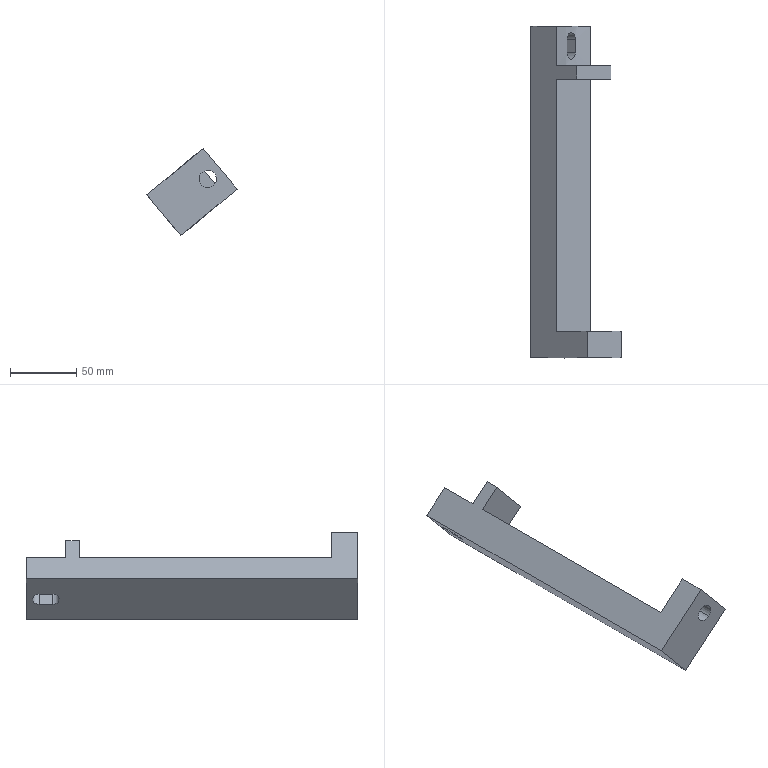Component | SolidWorks | K51-2_K51-5-2 | 1 solid | 18 faces | box 67.87 x 250 x 65.92 mm | volume 273386 mm3 | plane 13 | cylinder 5 | commonest cylinder face diameters 13 x2 10 x2 170 x1
build123d program:
from build123d import *

# Parameters (mm, degrees)
BOSS_EXTRUDE1_DEPTH = 20
SKETCH2_R           = 6.5
CUT_EXTRUDE1_DEPTH  = 30
SKETCH3_W           = 40
SKETCH3_H           = 10
BOSS_EXTRUDE2_DEPTH = 20
SKETCH4_R           = 85
CUT_EXTRUDE2_DEPTH  = 30
CUT_EXTRUDE3_DEPTH  = 30


with BuildPart() as part:
    # Sketch1 → Boss-Extrude1 (new, symmetric)
    with BuildSketch(Plane.XY):
        Polygon((0, 0), (0, 250), (25, 250), (25, 20), (55, 20), (55, 0), align=None)
    extrude(amount=BOSS_EXTRUDE1_DEPTH, both=True)

    # Sketch2 → Cut-Extrude1 (cut)
    with BuildSketch(Plane(origin=(0, 20, 0), x_dir=(1, 0, 0), z_dir=(0, 1, 0))):
        with Locations(Location((43, 0, 0), (0, 0, 270))):
            Circle(SKETCH2_R)
    extrude(amount=-CUT_EXTRUDE1_DEPTH, mode=Mode.SUBTRACT)

    # Sketch3 → Boss-Extrude2 (add)
    with BuildSketch(Plane(origin=(25, 0, 0), x_dir=(0, 0, -1), z_dir=(1, 0, 0))):
        with Locations((0, 215)):
            Rectangle(SKETCH3_W, SKETCH3_H)
    extrude(amount=BOSS_EXTRUDE2_DEPTH)

    # Sketch4 → Cut-Extrude2 (cut)
    with BuildSketch(Plane(origin=(0, 250, 0), x_dir=(1, 0, 0), z_dir=(0, 1, 0))):
        with Locations((107.614, 0)):
            Circle(SKETCH4_R)
    extrude(amount=-CUT_EXTRUDE2_DEPTH, mode=Mode.SUBTRACT)

    # Sketch5 → Cut-Extrude3 (cut)
    with BuildSketch(Plane.ZY):
        with BuildLine():
            Line((5, 240), (5, 230))
            ThreePointArc((5, 230), (0, 225), (-5, 230))
            Line((-5, 230), (-5, 240))
            ThreePointArc((-5, 240), (0, 245), (5, 240))
        make_face()
    extrude(amount=-CUT_EXTRUDE3_DEPTH, mode=Mode.SUBTRACT)


solid = part.part

# Placed as in the assembly
solid = solid.moved(Location((-338.347, 1052, 8.26), (0, -39.731, 0)))
STEP:
#1=COLOUR_RGB('',0.7922,0.8196,0.9333);
#2=FILL_AREA_STYLE_COLOUR('',#1);
#3=FILL_AREA_STYLE('',(#2));
#4=SURFACE_STYLE_FILL_AREA(#3);
#5=SURFACE_SIDE_STYLE('',(#4));
#6=SURFACE_STYLE_USAGE(.BOTH.,#5);
#7=PRESENTATION_STYLE_ASSIGNMENT((#6));
#8=CARTESIAN_POINT('',(-11.855,41.417,1.21));
#9=VERTEX_POINT('',#8);
#10=CARTESIAN_POINT('',(-12.182,41.417,1.604));
#11=VERTEX_POINT('',#10);
#12=CARTESIAN_POINT('',(-12.019,41.417,1.407));
#13=DIRECTION('',(-0.,1.,-0.));
#14=DIRECTION('',(-0.769,0.,-0.6392));
#15=AXIS2_PLACEMENT_3D('',#12,#13,#14);
#16=CIRCLE('',#15,0.2559);
#17=EDGE_CURVE('',#9,#11,#16,.T.);
#18=ORIENTED_EDGE('',*,*,#17,.F.);
#19=CARTESIAN_POINT('',(-11.855,42.205,1.21));
#20=VERTEX_POINT('',#19);
#21=CARTESIAN_POINT('',(-11.855,41.024,1.21));
#22=DIRECTION('',(-0.,1.,-0.));
#23=VECTOR('',#22,39.37);
#24=LINE('',#21,#23);
#25=EDGE_CURVE('',#9,#20,#24,.T.);
#26=ORIENTED_EDGE('',*,*,#25,.T.);
#27=CARTESIAN_POINT('',(-12.182,42.205,1.604));
#28=VERTEX_POINT('',#27);
#29=CARTESIAN_POINT('',(-12.019,42.205,1.407));
#30=DIRECTION('',(-0.,1.,-0.));
#31=DIRECTION('',(-0.6392,0.,0.769));
#32=AXIS2_PLACEMENT_3D('',#29,#30,#31);
#33=CIRCLE('',#32,0.2559);
#34=EDGE_CURVE('',#20,#28,#33,.T.);
#35=ORIENTED_EDGE('',*,*,#34,.T.);
#36=CARTESIAN_POINT('',(-12.182,41.024,1.604));
#37=DIRECTION('',(-0.,1.,-0.));
#38=VECTOR('',#37,39.37);
#39=LINE('',#36,#38);
#40=EDGE_CURVE('',#11,#28,#39,.T.);
#41=ORIENTED_EDGE('',*,*,#40,.F.);
#42=EDGE_LOOP('',(#18,#26,#35,#41));
#43=FACE_OUTER_BOUND('',#42,.T.);
#44=CARTESIAN_POINT('',(-12.019,41.024,1.407));
#45=DIRECTION('',(-0.,1.,-0.));
#46=DIRECTION('',(-0.6392,0.,0.769));
#47=AXIS2_PLACEMENT_3D('',#44,#45,#46);
#48=CYLINDRICAL_SURFACE('',#47,0.2559);
#49=ADVANCED_FACE('',(#43),#48,.F.);
#50=CARTESIAN_POINT('',(-13.067,49.685,1.56));
#51=VERTEX_POINT('',#50);
#52=CARTESIAN_POINT('',(-12.061,49.685,0.3487));
#53=VERTEX_POINT('',#52);
#54=CARTESIAN_POINT('',(-13.067,49.685,1.56));
#55=DIRECTION('',(0.6392,-0.,-0.769));
#56=VECTOR('',#55,39.37);
#57=LINE('',#54,#56);
#58=EDGE_CURVE('',#51,#53,#57,.T.);
#59=ORIENTED_EDGE('',*,*,#58,.F.);
#60=CARTESIAN_POINT('',(-13.067,42.205,1.56));
#61=VERTEX_POINT('',#60);
#62=CARTESIAN_POINT('',(-13.067,51.26,1.56));
#63=DIRECTION('',(-0.,1.,-0.));
#64=VECTOR('',#63,39.37);
#65=LINE('',#62,#64);
#66=EDGE_CURVE('',#61,#51,#65,.T.);
#67=ORIENTED_EDGE('',*,*,#66,.F.);
#68=CARTESIAN_POINT('',(-12.061,42.205,0.3487));
#69=VERTEX_POINT('',#68);
#70=CARTESIAN_POINT('',(-13.067,42.205,1.56));
#71=DIRECTION('',(0.6392,-0.,-0.769));
#72=VECTOR('',#71,39.37);
#73=LINE('',#70,#72);
#74=EDGE_CURVE('',#61,#69,#73,.T.);
#75=ORIENTED_EDGE('',*,*,#74,.T.);
#76=CARTESIAN_POINT('',(-12.061,51.26,0.3487));
#77=DIRECTION('',(-0.,1.,-0.));
#78=VECTOR('',#77,39.37);
#79=LINE('',#76,#78);
#80=EDGE_CURVE('',#69,#53,#79,.T.);
#81=ORIENTED_EDGE('',*,*,#80,.T.);
#82=EDGE_LOOP('',(#59,#67,#75,#81));
#83=FACE_OUTER_BOUND('',#82,.T.);
#84=CARTESIAN_POINT('',(-13.067,51.26,1.56));
#85=DIRECTION('',(-0.769,-0.,-0.6392));
#86=DIRECTION('',(0.,-1.,0.));
#87=AXIS2_PLACEMENT_3D('',#84,#85,#86);
#88=PLANE('',#87);
#89=ADVANCED_FACE('',(#83),#88,.F.);
#90=CARTESIAN_POINT('',(-12.019,41.417,1.407));
#91=DIRECTION('',(-0.,1.,-0.));
#92=DIRECTION('',(-0.769,0.,-0.6392));
#93=AXIS2_PLACEMENT_3D('',#90,#91,#92);
#94=CIRCLE('',#93,0.2559);
#95=EDGE_CURVE('',#11,#9,#94,.T.);
#96=ORIENTED_EDGE('',*,*,#95,.T.);
#97=ORIENTED_EDGE('',*,*,#17,.T.);
#98=EDGE_LOOP('',(#96,#97));
#99=FACE_BOUND('',#98,.T.);
#100=CARTESIAN_POINT('',(-12.817,41.417,-0.2804));
#101=VERTEX_POINT('',#100);
#102=CARTESIAN_POINT('',(-11.152,41.417,1.104));
#103=VERTEX_POINT('',#102);
#104=CARTESIAN_POINT('',(-11.152,41.417,1.104));
#105=DIRECTION('',(0.769,0.,0.6392));
#106=VECTOR('',#105,39.37);
#107=LINE('',#104,#106);
#108=EDGE_CURVE('',#101,#103,#107,.T.);
#109=ORIENTED_EDGE('',*,*,#108,.T.);
#110=CARTESIAN_POINT('',(-12.159,41.417,2.315));
#111=VERTEX_POINT('',#110);
#112=CARTESIAN_POINT('',(-12.159,41.417,2.315));
#113=DIRECTION('',(0.6392,-0.,-0.769));
#114=VECTOR('',#113,39.37);
#115=LINE('',#112,#114);
#116=EDGE_CURVE('',#111,#103,#115,.T.);
#117=ORIENTED_EDGE('',*,*,#116,.F.);
#118=CARTESIAN_POINT('',(-13.824,41.417,0.9307));
#119=VERTEX_POINT('',#118);
#120=CARTESIAN_POINT('',(-12.159,41.417,2.315));
#121=DIRECTION('',(0.769,0.,0.6392));
#122=VECTOR('',#121,39.37);
#123=LINE('',#120,#122);
#124=EDGE_CURVE('',#119,#111,#123,.T.);
#125=ORIENTED_EDGE('',*,*,#124,.F.);
#126=CARTESIAN_POINT('',(-13.824,41.417,0.9307));
#127=DIRECTION('',(0.6392,-0.,-0.769));
#128=VECTOR('',#127,39.37);
#129=LINE('',#126,#128);
#130=EDGE_CURVE('',#119,#101,#129,.T.);
#131=ORIENTED_EDGE('',*,*,#130,.T.);
#132=EDGE_LOOP('',(#109,#117,#125,#131));
#133=FACE_OUTER_BOUND('',#132,.T.);
#134=CARTESIAN_POINT('',(-12.159,41.417,2.315));
#135=DIRECTION('',(-0.,1.,-0.));
#136=DIRECTION('',(-0.769,-0.,-0.6392));
#137=AXIS2_PLACEMENT_3D('',#134,#135,#136);
#138=PLANE('',#137);
#139=ADVANCED_FACE('',(#99,#133),#138,.F.);
#140=CARTESIAN_POINT('',(-11.152,42.205,1.104));
#141=VERTEX_POINT('',#140);
#142=CARTESIAN_POINT('',(-11.152,42.205,1.104));
#143=DIRECTION('',(-0.,1.,-0.));
#144=VECTOR('',#143,39.37);
#145=LINE('',#142,#144);
#146=EDGE_CURVE('',#103,#141,#145,.T.);
#147=ORIENTED_EDGE('',*,*,#146,.T.);
#148=CARTESIAN_POINT('',(-12.159,42.205,2.315));
#149=VERTEX_POINT('',#148);
#150=CARTESIAN_POINT('',(-12.159,42.205,2.315));
#151=DIRECTION('',(0.6392,-0.,-0.769));
#152=VECTOR('',#151,39.37);
#153=LINE('',#150,#152);
#154=EDGE_CURVE('',#149,#141,#153,.T.);
#155=ORIENTED_EDGE('',*,*,#154,.F.);
#156=CARTESIAN_POINT('',(-12.159,42.205,2.315));
#157=DIRECTION('',(-0.,1.,-0.));
#158=VECTOR('',#157,39.37);
#159=LINE('',#156,#158);
#160=EDGE_CURVE('',#111,#149,#159,.T.);
#161=ORIENTED_EDGE('',*,*,#160,.F.);
#162=ORIENTED_EDGE('',*,*,#116,.T.);
#163=EDGE_LOOP('',(#147,#155,#161,#162));
#164=FACE_OUTER_BOUND('',#163,.T.);
#165=CARTESIAN_POINT('',(-12.159,42.205,2.315));
#166=DIRECTION('',(-0.769,-0.,-0.6392));
#167=DIRECTION('',(-0.6392,0.,0.769));
#168=AXIS2_PLACEMENT_3D('',#165,#166,#167);
#169=PLANE('',#168);
#170=ADVANCED_FACE('',(#164),#169,.F.);
#171=CARTESIAN_POINT('',(-12.019,42.205,1.407));
#172=DIRECTION('',(-0.,1.,-0.));
#173=DIRECTION('',(-0.6392,0.,0.769));
#174=AXIS2_PLACEMENT_3D('',#171,#172,#173);
#175=CIRCLE('',#174,0.2559);
#176=EDGE_CURVE('',#28,#20,#175,.T.);
#177=ORIENTED_EDGE('',*,*,#176,.F.);
#178=ORIENTED_EDGE('',*,*,#34,.F.);
#179=EDGE_LOOP('',(#177,#178));
#180=FACE_BOUND('',#179,.T.);
#181=CARTESIAN_POINT('',(-12.061,42.205,0.3487));
#182=DIRECTION('',(-0.769,-0.,-0.6392));
#183=VECTOR('',#182,39.37);
#184=LINE('',#181,#183);
#185=EDGE_CURVE('',#141,#69,#184,.T.);
#186=ORIENTED_EDGE('',*,*,#185,.T.);
#187=ORIENTED_EDGE('',*,*,#74,.F.);
#188=CARTESIAN_POINT('',(-13.067,42.205,1.56));
#189=DIRECTION('',(-0.769,-0.,-0.6392));
#190=VECTOR('',#189,39.37);
#191=LINE('',#188,#190);
#192=EDGE_CURVE('',#149,#61,#191,.T.);
#193=ORIENTED_EDGE('',*,*,#192,.F.);
#194=ORIENTED_EDGE('',*,*,#154,.T.);
#195=EDGE_LOOP('',(#186,#187,#193,#194));
#196=FACE_OUTER_BOUND('',#195,.T.);
#197=CARTESIAN_POINT('',(-13.067,42.205,1.56));
#198=DIRECTION('',(0.,-1.,0.));
#199=DIRECTION('',(0.6392,-0.,-0.769));
#200=AXIS2_PLACEMENT_3D('',#197,#198,#199);
#201=PLANE('',#200);
#202=ADVANCED_FACE('',(#180,#196),#201,.F.);
#203=CARTESIAN_POINT('',(-13.067,51.26,1.56));
#204=VERTEX_POINT('',#203);
#205=CARTESIAN_POINT('',(-13.824,51.26,0.9307));
#206=VERTEX_POINT('',#205);
#207=CARTESIAN_POINT('',(-13.824,51.26,0.9307));
#208=DIRECTION('',(-0.769,-0.,-0.6392));
#209=VECTOR('',#208,39.37);
#210=LINE('',#207,#209);
#211=EDGE_CURVE('',#204,#206,#210,.T.);
#212=ORIENTED_EDGE('',*,*,#211,.F.);
#213=CARTESIAN_POINT('',(-12.061,51.26,0.3487));
#214=VERTEX_POINT('',#213);
#215=CARTESIAN_POINT('',(-10.062,51.26,3.033));
#216=DIRECTION('',(-0.,1.,-0.));
#217=DIRECTION('',(-0.6392,0.,0.769));
#218=AXIS2_PLACEMENT_3D('',#215,#216,#217);
#219=CIRCLE('',#218,3.346);
#220=EDGE_CURVE('',#214,#204,#219,.T.);
#221=ORIENTED_EDGE('',*,*,#220,.F.);
#222=CARTESIAN_POINT('',(-12.817,51.26,-0.2804));
#223=VERTEX_POINT('',#222);
#224=CARTESIAN_POINT('',(-12.817,51.26,-0.2804));
#225=DIRECTION('',(-0.769,-0.,-0.6392));
#226=VECTOR('',#225,39.37);
#227=LINE('',#224,#226);
#228=EDGE_CURVE('',#214,#223,#227,.T.);
#229=ORIENTED_EDGE('',*,*,#228,.T.);
#230=CARTESIAN_POINT('',(-13.824,51.26,0.9307));
#231=DIRECTION('',(0.6392,-0.,-0.769));
#232=VECTOR('',#231,39.37);
#233=LINE('',#230,#232);
#234=EDGE_CURVE('',#206,#223,#233,.T.);
#235=ORIENTED_EDGE('',*,*,#234,.F.);
#236=EDGE_LOOP('',(#212,#221,#229,#235));
#237=FACE_OUTER_BOUND('',#236,.T.);
#238=CARTESIAN_POINT('',(-13.824,51.26,0.9307));
#239=DIRECTION('',(0.,-1.,0.));
#240=DIRECTION('',(0.6392,-0.,-0.769));
#241=AXIS2_PLACEMENT_3D('',#238,#239,#240);
#242=PLANE('',#241);
#243=ADVANCED_FACE('',(#237),#242,.F.);
#244=CARTESIAN_POINT('',(-13.195,50.866,0.1738));
#245=VERTEX_POINT('',#244);
#246=CARTESIAN_POINT('',(-13.195,50.472,0.1738));
#247=VERTEX_POINT('',#246);
#248=CARTESIAN_POINT('',(-13.195,50.866,0.1738));
#249=DIRECTION('',(0.,-1.,0.));
#250=VECTOR('',#249,39.37);
#251=LINE('',#248,#250);
#252=EDGE_CURVE('',#245,#247,#251,.T.);
#253=ORIENTED_EDGE('',*,*,#252,.F.);
#254=CARTESIAN_POINT('',(-13.447,50.866,0.4766));
#255=VERTEX_POINT('',#254);
#256=CARTESIAN_POINT('',(-13.321,50.866,0.3252));
#257=DIRECTION('',(-0.769,-0.,-0.6392));
#258=DIRECTION('',(-0.6392,0.,0.769));
#259=AXIS2_PLACEMENT_3D('',#256,#257,#258);
#260=CIRCLE('',#259,0.1969);
#261=EDGE_CURVE('',#255,#245,#260,.T.);
#262=ORIENTED_EDGE('',*,*,#261,.F.);
#263=CARTESIAN_POINT('',(-13.447,50.472,0.4766));
#264=VERTEX_POINT('',#263);
#265=CARTESIAN_POINT('',(-13.447,50.866,0.4766));
#266=DIRECTION('',(-0.,1.,-0.));
#267=VECTOR('',#266,39.37);
#268=LINE('',#265,#267);
#269=EDGE_CURVE('',#264,#255,#268,.T.);
#270=ORIENTED_EDGE('',*,*,#269,.F.);
#271=CARTESIAN_POINT('',(-13.321,50.472,0.3252));
#272=DIRECTION('',(-0.769,-0.,-0.6392));
#273=DIRECTION('',(-0.6392,0.,0.769));
#274=AXIS2_PLACEMENT_3D('',#271,#272,#273);
#275=CIRCLE('',#274,0.1969);
#276=EDGE_CURVE('',#247,#264,#275,.T.);
#277=ORIENTED_EDGE('',*,*,#276,.F.);
#278=EDGE_LOOP('',(#253,#262,#270,#277));
#279=FACE_BOUND('',#278,.T.);
#280=CARTESIAN_POINT('',(-12.817,41.417,-0.2804));
#281=DIRECTION('',(0.,-1.,0.));
#282=VECTOR('',#281,39.37);
#283=LINE('',#280,#282);
#284=EDGE_CURVE('',#223,#101,#283,.T.);
#285=ORIENTED_EDGE('',*,*,#284,.T.);
#286=ORIENTED_EDGE('',*,*,#130,.F.);
#287=CARTESIAN_POINT('',(-13.824,41.417,0.9307));
#288=DIRECTION('',(0.,-1.,0.));
#289=VECTOR('',#288,39.37);
#290=LINE('',#287,#289);
#291=EDGE_CURVE('',#206,#119,#290,.T.);
#292=ORIENTED_EDGE('',*,*,#291,.F.);
#293=ORIENTED_EDGE('',*,*,#234,.T.);
#294=EDGE_LOOP('',(#285,#286,#292,#293));
#295=FACE_OUTER_BOUND('',#294,.T.);
#296=CARTESIAN_POINT('',(-13.824,41.417,0.9307));
#297=DIRECTION('',(0.769,0.,0.6392));
#298=DIRECTION('',(0.6392,-0.,-0.769));
#299=AXIS2_PLACEMENT_3D('',#296,#297,#298);
#300=PLANE('',#299);
#301=ADVANCED_FACE('',(#279,#295),#300,.F.);
#302=ORIENTED_EDGE('',*,*,#124,.T.);
#303=ORIENTED_EDGE('',*,*,#160,.T.);
#304=ORIENTED_EDGE('',*,*,#192,.T.);
#305=ORIENTED_EDGE('',*,*,#66,.T.);
#306=CARTESIAN_POINT('',(-12.462,49.685,2.063));
#307=VERTEX_POINT('',#306);
#308=CARTESIAN_POINT('',(-12.462,49.685,2.063));
#309=DIRECTION('',(-0.769,-0.,-0.6392));
#310=VECTOR('',#309,39.37);
#311=LINE('',#308,#310);
#312=EDGE_CURVE('',#307,#51,#311,.T.);
#313=ORIENTED_EDGE('',*,*,#312,.F.);
#314=CARTESIAN_POINT('',(-12.462,50.079,2.063));
#315=VERTEX_POINT('',#314);
#316=CARTESIAN_POINT('',(-12.462,50.079,2.063));
#317=DIRECTION('',(0.,-1.,0.));
#318=VECTOR('',#317,39.37);
#319=LINE('',#316,#318);
#320=EDGE_CURVE('',#315,#307,#319,.T.);
#321=ORIENTED_EDGE('',*,*,#320,.F.);
#322=CARTESIAN_POINT('',(-13.067,50.079,1.56));
#323=VERTEX_POINT('',#322);
#324=CARTESIAN_POINT('',(-12.462,50.079,2.063));
#325=DIRECTION('',(-0.769,-0.,-0.6392));
#326=VECTOR('',#325,39.37);
#327=LINE('',#324,#326);
#328=EDGE_CURVE('',#315,#323,#327,.T.);
#329=ORIENTED_EDGE('',*,*,#328,.T.);
#330=CARTESIAN_POINT('',(-13.067,51.26,1.56));
#331=DIRECTION('',(-0.,1.,-0.));
#332=VECTOR('',#331,39.37);
#333=LINE('',#330,#332);
#334=EDGE_CURVE('',#323,#204,#333,.T.);
#335=ORIENTED_EDGE('',*,*,#334,.T.);
#336=ORIENTED_EDGE('',*,*,#211,.T.);
#337=ORIENTED_EDGE('',*,*,#291,.T.);
#338=EDGE_LOOP('',(#302,#303,#304,#305,#313,#321,#329,#335,#336,#337));
#339=FACE_OUTER_BOUND('',#338,.T.);
#340=CARTESIAN_POINT('',(-13.824,41.417,0.9307));
#341=DIRECTION('',(0.6392,-0.,-0.769));
#342=DIRECTION('',(-0.769,-0.,-0.6392));
#343=AXIS2_PLACEMENT_3D('',#340,#341,#342);
#344=PLANE('',#343);
#345=ADVANCED_FACE('',(#339),#344,.F.);
#346=ORIENTED_EDGE('',*,*,#108,.F.);
#347=ORIENTED_EDGE('',*,*,#284,.F.);
#348=ORIENTED_EDGE('',*,*,#228,.F.);
#349=CARTESIAN_POINT('',(-12.061,50.079,0.3487));
#350=VERTEX_POINT('',#349);
#351=CARTESIAN_POINT('',(-12.061,51.26,0.3487));
#352=DIRECTION('',(-0.,1.,-0.));
#353=VECTOR('',#352,39.37);
#354=LINE('',#351,#353);
#355=EDGE_CURVE('',#350,#214,#354,.T.);
#356=ORIENTED_EDGE('',*,*,#355,.F.);
#357=CARTESIAN_POINT('',(-11.455,50.079,0.852));
#358=VERTEX_POINT('',#357);
#359=CARTESIAN_POINT('',(-11.455,50.079,0.852));
#360=DIRECTION('',(-0.769,-0.,-0.6392));
#361=VECTOR('',#360,39.37);
#362=LINE('',#359,#361);
#363=EDGE_CURVE('',#358,#350,#362,.T.);
#364=ORIENTED_EDGE('',*,*,#363,.F.);
#365=CARTESIAN_POINT('',(-11.455,49.685,0.852));
#366=VERTEX_POINT('',#365);
#367=CARTESIAN_POINT('',(-11.455,50.079,0.852));
#368=DIRECTION('',(-0.,1.,-0.));
#369=VECTOR('',#368,39.37);
#370=LINE('',#367,#369);
#371=EDGE_CURVE('',#366,#358,#370,.T.);
#372=ORIENTED_EDGE('',*,*,#371,.F.);
#373=CARTESIAN_POINT('',(-11.455,49.685,0.852));
#374=DIRECTION('',(-0.769,-0.,-0.6392));
#375=VECTOR('',#374,39.37);
#376=LINE('',#373,#375);
#377=EDGE_CURVE('',#366,#53,#376,.T.);
#378=ORIENTED_EDGE('',*,*,#377,.T.);
#379=ORIENTED_EDGE('',*,*,#80,.F.);
#380=ORIENTED_EDGE('',*,*,#185,.F.);
#381=ORIENTED_EDGE('',*,*,#146,.F.);
#382=EDGE_LOOP('',(#346,#347,#348,#356,#364,#372,#378,#379,#380,#381));
#383=FACE_OUTER_BOUND('',#382,.T.);
#384=CARTESIAN_POINT('',(-12.817,41.417,-0.2804));
#385=DIRECTION('',(0.6392,-0.,-0.769));
#386=DIRECTION('',(-0.769,-0.,-0.6392));
#387=AXIS2_PLACEMENT_3D('',#384,#385,#386);
#388=PLANE('',#387);
#389=ADVANCED_FACE('',(#383),#388,.T.);
#390=ORIENTED_EDGE('',*,*,#25,.F.);
#391=ORIENTED_EDGE('',*,*,#95,.F.);
#392=ORIENTED_EDGE('',*,*,#40,.T.);
#393=ORIENTED_EDGE('',*,*,#176,.T.);
#394=EDGE_LOOP('',(#390,#391,#392,#393));
#395=FACE_OUTER_BOUND('',#394,.T.);
#396=CARTESIAN_POINT('',(-12.019,41.024,1.407));
#397=DIRECTION('',(-0.,1.,-0.));
#398=DIRECTION('',(-0.6392,0.,0.769));
#399=AXIS2_PLACEMENT_3D('',#396,#397,#398);
#400=CYLINDRICAL_SURFACE('',#399,0.2559);
#401=ADVANCED_FACE('',(#395),#400,.F.);
#402=ORIENTED_EDGE('',*,*,#58,.T.);
#403=ORIENTED_EDGE('',*,*,#377,.F.);
#404=CARTESIAN_POINT('',(-12.462,49.685,2.063));
#405=DIRECTION('',(0.6392,-0.,-0.769));
#406=VECTOR('',#405,39.37);
#407=LINE('',#404,#406);
#408=EDGE_CURVE('',#307,#366,#407,.T.);
#409=ORIENTED_EDGE('',*,*,#408,.F.);
#410=ORIENTED_EDGE('',*,*,#312,.T.);
#411=EDGE_LOOP('',(#402,#403,#409,#410));
#412=FACE_OUTER_BOUND('',#411,.T.);
#413=CARTESIAN_POINT('',(-12.462,49.685,2.063));
#414=DIRECTION('',(-0.,1.,-0.));
#415=DIRECTION('',(-0.769,-0.,-0.6392));
#416=AXIS2_PLACEMENT_3D('',#413,#414,#415);
#417=PLANE('',#416);
#418=ADVANCED_FACE('',(#412),#417,.F.);
#419=ORIENTED_EDGE('',*,*,#363,.T.);
#420=CARTESIAN_POINT('',(-10.062,50.079,3.033));
#421=DIRECTION('',(-0.,1.,-0.));
#422=DIRECTION('',(0.769,0.,0.6392));
#423=AXIS2_PLACEMENT_3D('',#420,#421,#422);
#424=CIRCLE('',#423,3.346);
#425=EDGE_CURVE('',#350,#323,#424,.T.);
#426=ORIENTED_EDGE('',*,*,#425,.T.);
#427=ORIENTED_EDGE('',*,*,#328,.F.);
#428=CARTESIAN_POINT('',(-12.462,50.079,2.063));
#429=DIRECTION('',(-0.6392,0.,0.769));
#430=VECTOR('',#429,39.37);
#431=LINE('',#428,#430);
#432=EDGE_CURVE('',#358,#315,#431,.T.);
#433=ORIENTED_EDGE('',*,*,#432,.F.);
#434=EDGE_LOOP('',(#419,#426,#427,#433));
#435=FACE_OUTER_BOUND('',#434,.T.);
#436=CARTESIAN_POINT('',(-12.462,50.079,2.063));
#437=DIRECTION('',(0.,-1.,0.));
#438=DIRECTION('',(0.769,0.,0.6392));
#439=AXIS2_PLACEMENT_3D('',#436,#437,#438);
#440=PLANE('',#439);
#441=ADVANCED_FACE('',(#435),#440,.F.);
#442=ORIENTED_EDGE('',*,*,#320,.T.);
#443=ORIENTED_EDGE('',*,*,#408,.T.);
#444=ORIENTED_EDGE('',*,*,#371,.T.);
#445=ORIENTED_EDGE('',*,*,#432,.T.);
#446=EDGE_LOOP('',(#442,#443,#444,#445));
#447=FACE_OUTER_BOUND('',#446,.T.);
#448=CARTESIAN_POINT('',(-11.958,41.417,1.458));
#449=DIRECTION('',(0.769,0.,0.6392));
#450=DIRECTION('',(0.6392,-0.,-0.769));
#451=AXIS2_PLACEMENT_3D('',#448,#449,#450);
#452=PLANE('',#451);
#453=ADVANCED_FACE('',(#447),#452,.T.);
#454=CARTESIAN_POINT('',(-12.757,50.472,1.049));
#455=VERTEX_POINT('',#454);
#456=CARTESIAN_POINT('',(-12.757,50.866,1.049));
#457=VERTEX_POINT('',#456);
#458=CARTESIAN_POINT('',(-12.757,40.614,1.049));
#459=DIRECTION('',(-0.,1.,-0.));
#460=VECTOR('',#459,39.37);
#461=LINE('',#458,#460);
#462=EDGE_CURVE('',#455,#457,#461,.T.);
#463=ORIENTED_EDGE('',*,*,#462,.T.);
#464=CARTESIAN_POINT('',(-12.506,50.866,0.7466));
#465=VERTEX_POINT('',#464);
#466=CARTESIAN_POINT('',(-12.757,50.866,1.049));
#467=CARTESIAN_POINT('',(-12.757,50.879,1.049));
#468=CARTESIAN_POINT('',(-12.757,50.892,1.048));
#469=CARTESIAN_POINT('',(-12.754,50.911,1.045));
#470=CARTESIAN_POINT('',(-12.754,50.917,1.044));
#471=CARTESIAN_POINT('',(-12.751,50.929,1.041));
#472=CARTESIAN_POINT('',(-12.75,50.936,1.039));
#473=CARTESIAN_POINT('',(-12.746,50.953,1.033));
#474=CARTESIAN_POINT('',(-12.742,50.965,1.028));
#475=CARTESIAN_POINT('',(-12.733,50.986,1.017));
#476=CARTESIAN_POINT('',(-12.728,50.996,1.01));
#477=CARTESIAN_POINT('',(-12.717,51.014,0.9959));
#478=CARTESIAN_POINT('',(-12.711,51.023,0.9881));
#479=CARTESIAN_POINT('',(-12.698,51.037,0.9711));
#480=CARTESIAN_POINT('',(-12.691,51.043,0.9621));
#481=CARTESIAN_POINT('',(-12.676,51.053,0.9435));
#482=CARTESIAN_POINT('',(-12.668,51.057,0.9338));
#483=CARTESIAN_POINT('',(-12.652,51.062,0.9141));
#484=CARTESIAN_POINT('',(-12.644,51.063,0.9042));
#485=CARTESIAN_POINT('',(-12.628,51.063,0.8845));
#486=CARTESIAN_POINT('',(-12.62,51.062,0.8745));
#487=CARTESIAN_POINT('',(-12.603,51.057,0.8553));
#488=CARTESIAN_POINT('',(-12.595,51.053,0.846));
#489=CARTESIAN_POINT('',(-12.58,51.043,0.828));
#490=CARTESIAN_POINT('',(-12.572,51.037,0.8193));
#491=CARTESIAN_POINT('',(-12.558,51.023,0.8034));
#492=CARTESIAN_POINT('',(-12.551,51.015,0.7959));
#493=CARTESIAN_POINT('',(-12.539,50.996,0.7823));
#494=CARTESIAN_POINT('',(-12.533,50.986,0.7763));
#495=CARTESIAN_POINT('',(-12.526,50.97,0.7684));
#496=CARTESIAN_POINT('',(-12.524,50.965,0.7659));
#497=CARTESIAN_POINT('',(-12.52,50.953,0.7614));
#498=CARTESIAN_POINT('',(-12.518,50.948,0.7594));
#499=CARTESIAN_POINT('',(-12.513,50.93,0.7539));
#500=CARTESIAN_POINT('',(-12.51,50.917,0.7512));
#501=CARTESIAN_POINT('',(-12.507,50.892,0.7475));
#502=CARTESIAN_POINT('',(-12.506,50.879,0.7466));
#503=CARTESIAN_POINT('',(-12.506,50.866,0.7466));
#504=B_SPLINE_CURVE_WITH_KNOTS('',3,(#466,#467,#468,#469,#470,#471,#472,#473,#474,#475,#476,#477,#478,#479,#480,#481,#482,#483,#484,#485,#486,#487,#488,#489,#490,#491,#492,#493,#494,#495,#496,#497,#498,#499,#500,#501,#502,#503),.UNSPECIFIED.,.F.,.F.,(4,2,2,2,2,2,2,2,2,2,2,2,2,2,2,2,2,2,4),(0.,0.000977,0.001466,0.001954,0.002931,0.003908,0.004885,0.005862,0.006839,0.007816,0.008793,0.00977,0.01075,0.01172,0.0127,0.01319,0.01368,0.01466,0.01563),.UNSPECIFIED.);
#505=EDGE_CURVE('',#457,#465,#504,.T.);
#506=ORIENTED_EDGE('',*,*,#505,.T.);
#507=CARTESIAN_POINT('',(-12.506,50.472,0.7466));
#508=VERTEX_POINT('',#507);
#509=CARTESIAN_POINT('',(-12.506,40.614,0.7466));
#510=DIRECTION('',(0.,-1.,0.));
#511=VECTOR('',#510,39.37);
#512=LINE('',#509,#511);
#513=EDGE_CURVE('',#465,#508,#512,.T.);
#514=ORIENTED_EDGE('',*,*,#513,.T.);
#515=CARTESIAN_POINT('',(-12.506,50.472,0.7466));
#516=CARTESIAN_POINT('',(-12.506,50.459,0.7466));
#517=CARTESIAN_POINT('',(-12.507,50.447,0.7475));
#518=CARTESIAN_POINT('',(-12.509,50.428,0.7502));
#519=CARTESIAN_POINT('',(-12.51,50.422,0.7514));
#520=CARTESIAN_POINT('',(-12.513,50.409,0.7541));
#521=CARTESIAN_POINT('',(-12.514,50.403,0.7557));
#522=CARTESIAN_POINT('',(-12.519,50.385,0.7612));
#523=CARTESIAN_POINT('',(-12.524,50.374,0.7656));
#524=CARTESIAN_POINT('',(-12.533,50.352,0.7762));
#525=CARTESIAN_POINT('',(-12.539,50.342,0.7823));
#526=CARTESIAN_POINT('',(-12.551,50.324,0.7958));
#527=CARTESIAN_POINT('',(-12.558,50.316,0.8032));
#528=CARTESIAN_POINT('',(-12.572,50.302,0.8193));
#529=CARTESIAN_POINT('',(-12.579,50.296,0.8279));
#530=CARTESIAN_POINT('',(-12.595,50.286,0.8457));
#531=CARTESIAN_POINT('',(-12.603,50.282,0.8551));
#532=CARTESIAN_POINT('',(-12.62,50.277,0.8745));
#533=CARTESIAN_POINT('',(-12.628,50.276,0.8843));
#534=CARTESIAN_POINT('',(-12.644,50.276,0.904));
#535=CARTESIAN_POINT('',(-12.652,50.277,0.9141));
#536=CARTESIAN_POINT('',(-12.668,50.282,0.9337));
#537=CARTESIAN_POINT('',(-12.676,50.286,0.9433));
#538=CARTESIAN_POINT('',(-12.691,50.295,0.9619));
#539=CARTESIAN_POINT('',(-12.698,50.302,0.971));
#540=CARTESIAN_POINT('',(-12.711,50.316,0.9879));
#541=CARTESIAN_POINT('',(-12.717,50.324,0.9958));
#542=CARTESIAN_POINT('',(-12.728,50.342,1.01));
#543=CARTESIAN_POINT('',(-12.733,50.352,1.017));
#544=CARTESIAN_POINT('',(-12.74,50.368,1.025));
#545=CARTESIAN_POINT('',(-12.742,50.374,1.028));
#546=CARTESIAN_POINT('',(-12.745,50.385,1.033));
#547=CARTESIAN_POINT('',(-12.747,50.391,1.035));
#548=CARTESIAN_POINT('',(-12.751,50.409,1.041));
#549=CARTESIAN_POINT('',(-12.754,50.421,1.044));
#550=CARTESIAN_POINT('',(-12.757,50.446,1.048));
#551=CARTESIAN_POINT('',(-12.757,50.459,1.049));
#552=CARTESIAN_POINT('',(-12.757,50.472,1.049));
#553=B_SPLINE_CURVE_WITH_KNOTS('',3,(#515,#516,#517,#518,#519,#520,#521,#522,#523,#524,#525,#526,#527,#528,#529,#530,#531,#532,#533,#534,#535,#536,#537,#538,#539,#540,#541,#542,#543,#544,#545,#546,#547,#548,#549,#550,#551,#552),.UNSPECIFIED.,.F.,.F.,(4,2,2,2,2,2,2,2,2,2,2,2,2,2,2,2,2,2,4),(0.,0.000977,0.001466,0.001954,0.002931,0.003908,0.004885,0.005862,0.006839,0.007816,0.008793,0.00977,0.01075,0.01172,0.0127,0.01319,0.01368,0.01466,0.01563),.UNSPECIFIED.);
#554=EDGE_CURVE('',#508,#455,#553,.T.);
#555=ORIENTED_EDGE('',*,*,#554,.T.);
#556=EDGE_LOOP('',(#463,#506,#514,#555));
#557=FACE_BOUND('',#556,.T.);
#558=ORIENTED_EDGE('',*,*,#425,.F.);
#559=ORIENTED_EDGE('',*,*,#355,.T.);
#560=ORIENTED_EDGE('',*,*,#220,.T.);
#561=ORIENTED_EDGE('',*,*,#334,.F.);
#562=EDGE_LOOP('',(#558,#559,#560,#561));
#563=FACE_OUTER_BOUND('',#562,.T.);
#564=CARTESIAN_POINT('',(-10.062,40.614,3.033));
#565=DIRECTION('',(-0.,1.,-0.));
#566=DIRECTION('',(-0.6392,0.,0.769));
#567=AXIS2_PLACEMENT_3D('',#564,#565,#566);
#568=CYLINDRICAL_SURFACE('',#567,3.346);
#569=ADVANCED_FACE('',(#557,#563),#568,.F.);
#570=CARTESIAN_POINT('',(-12.538,50.866,1.232));
#571=DIRECTION('',(-0.769,-0.,-0.6392));
#572=VECTOR('',#571,39.37);
#573=LINE('',#570,#572);
#574=EDGE_CURVE('',#457,#255,#573,.T.);
#575=ORIENTED_EDGE('',*,*,#574,.T.);
#576=ORIENTED_EDGE('',*,*,#261,.T.);
#577=CARTESIAN_POINT('',(-12.287,50.866,0.9287));
#578=DIRECTION('',(-0.769,-0.,-0.6392));
#579=VECTOR('',#578,39.37);
#580=LINE('',#577,#579);
#581=EDGE_CURVE('',#465,#245,#580,.T.);
#582=ORIENTED_EDGE('',*,*,#581,.F.);
#583=ORIENTED_EDGE('',*,*,#505,.F.);
#584=EDGE_LOOP('',(#575,#576,#582,#583));
#585=FACE_OUTER_BOUND('',#584,.T.);
#586=CARTESIAN_POINT('',(-12.412,50.866,1.08));
#587=DIRECTION('',(-0.769,-0.,-0.6392));
#588=DIRECTION('',(-0.6392,0.,0.769));
#589=AXIS2_PLACEMENT_3D('',#586,#587,#588);
#590=CYLINDRICAL_SURFACE('',#589,0.1969);
#591=ADVANCED_FACE('',(#585),#590,.F.);
#592=CARTESIAN_POINT('',(-12.538,50.472,1.232));
#593=DIRECTION('',(-0.769,-0.,-0.6392));
#594=VECTOR('',#593,39.37);
#595=LINE('',#592,#594);
#596=EDGE_CURVE('',#455,#264,#595,.T.);
#597=ORIENTED_EDGE('',*,*,#596,.T.);
#598=ORIENTED_EDGE('',*,*,#269,.T.);
#599=ORIENTED_EDGE('',*,*,#574,.F.);
#600=ORIENTED_EDGE('',*,*,#462,.F.);
#601=EDGE_LOOP('',(#597,#598,#599,#600));
#602=FACE_OUTER_BOUND('',#601,.T.);
#603=CARTESIAN_POINT('',(-12.538,50.866,1.232));
#604=DIRECTION('',(-0.6392,0.,0.769));
#605=DIRECTION('',(0.,-1.,0.));
#606=AXIS2_PLACEMENT_3D('',#603,#604,#605);
#607=PLANE('',#606);
#608=ADVANCED_FACE('',(#602),#607,.F.);
#609=CARTESIAN_POINT('',(-12.287,50.472,0.9287));
#610=DIRECTION('',(-0.769,-0.,-0.6392));
#611=VECTOR('',#610,39.37);
#612=LINE('',#609,#611);
#613=EDGE_CURVE('',#508,#247,#612,.T.);
#614=ORIENTED_EDGE('',*,*,#613,.T.);
#615=ORIENTED_EDGE('',*,*,#276,.T.);
#616=ORIENTED_EDGE('',*,*,#596,.F.);
#617=ORIENTED_EDGE('',*,*,#554,.F.);
#618=EDGE_LOOP('',(#614,#615,#616,#617));
#619=FACE_OUTER_BOUND('',#618,.T.);
#620=CARTESIAN_POINT('',(-12.412,50.472,1.08));
#621=DIRECTION('',(-0.769,-0.,-0.6392));
#622=DIRECTION('',(-0.6392,0.,0.769));
#623=AXIS2_PLACEMENT_3D('',#620,#621,#622);
#624=CYLINDRICAL_SURFACE('',#623,0.1969);
#625=ADVANCED_FACE('',(#619),#624,.F.);
#626=ORIENTED_EDGE('',*,*,#581,.T.);
#627=ORIENTED_EDGE('',*,*,#252,.T.);
#628=ORIENTED_EDGE('',*,*,#613,.F.);
#629=ORIENTED_EDGE('',*,*,#513,.F.);
#630=EDGE_LOOP('',(#626,#627,#628,#629));
#631=FACE_OUTER_BOUND('',#630,.T.);
#632=CARTESIAN_POINT('',(-12.287,50.866,0.9287));
#633=DIRECTION('',(0.6392,-0.,-0.769));
#634=DIRECTION('',(-0.,1.,-0.));
#635=AXIS2_PLACEMENT_3D('',#632,#633,#634);
#636=PLANE('',#635);
#637=ADVANCED_FACE('',(#631),#636,.F.);
#638=CLOSED_SHELL('',(#49,#89,#139,#170,#202,#243,#301,#345,#389,#401,#418,#441,#453,#569,#591,#608,#625,#637));
#639=MANIFOLD_SOLID_BREP('',#638);
#640=STYLED_ITEM('',(#7),#639);
#641=PRESENTATION_LAYER_ASSIGNMENT('','',(#640));
#642=CARTESIAN_POINT('',(0.,0.,0.));
#643=DIRECTION('',(0.,0.,1.));
#644=DIRECTION('',(1.,0.,0.));
#645=AXIS2_PLACEMENT_3D('',#642,#643,#644);
#646=(LENGTH_UNIT()NAMED_UNIT(*)SI_UNIT($,.METRE.));
#647=LENGTH_MEASURE_WITH_UNIT(LENGTH_MEASURE(0.0254),#646);
#648=DIMENSIONAL_EXPONENTS(1.,0.,0.,0.,0.,0.,0.);
#649=(CONVERSION_BASED_UNIT('',#647)LENGTH_UNIT()NAMED_UNIT(#648));
#650=UNCERTAINTY_MEASURE_WITH_UNIT(LENGTH_MEASURE(0.00001),#649,'','');
#651=(NAMED_UNIT(*)PLANE_ANGLE_UNIT()SI_UNIT($,.RADIAN.));
#652=(NAMED_UNIT(*)SI_UNIT($,.STERADIAN.)SOLID_ANGLE_UNIT());
#653=(GEOMETRIC_REPRESENTATION_CONTEXT(3)GLOBAL_UNCERTAINTY_ASSIGNED_CONTEXT((#650))GLOBAL_UNIT_ASSIGNED_CONTEXT((#649,#651,#652))REPRESENTATION_CONTEXT('',''));
#654=ADVANCED_BREP_SHAPE_REPRESENTATION('',(#639,#645),#653);
#655=(LENGTH_UNIT()NAMED_UNIT(*)SI_UNIT($,.METRE.));
#656=LENGTH_MEASURE_WITH_UNIT(LENGTH_MEASURE(0.0254),#655);
#657=DIMENSIONAL_EXPONENTS(1.,0.,0.,0.,0.,0.,0.);
#658=(CONVERSION_BASED_UNIT('',#656)LENGTH_UNIT()NAMED_UNIT(#657));
#659=UNCERTAINTY_MEASURE_WITH_UNIT(LENGTH_MEASURE(0.00001),#658,'','');
#660=(NAMED_UNIT(*)PLANE_ANGLE_UNIT()SI_UNIT($,.RADIAN.));
#661=(NAMED_UNIT(*)SI_UNIT($,.STERADIAN.)SOLID_ANGLE_UNIT());
#662=(GEOMETRIC_REPRESENTATION_CONTEXT(3)GLOBAL_UNCERTAINTY_ASSIGNED_CONTEXT((#659))GLOBAL_UNIT_ASSIGNED_CONTEXT((#658,#660,#661))REPRESENTATION_CONTEXT('',''));
#663=MECHANICAL_DESIGN_GEOMETRIC_PRESENTATION_REPRESENTATION('',(#640),#662);